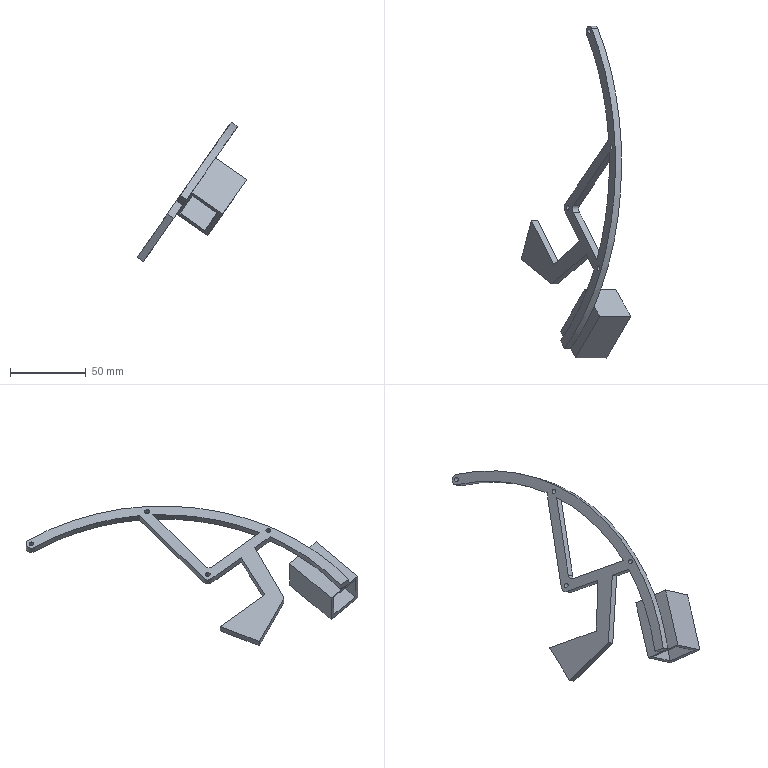Component | NX | LOWER_LEG | 1 solid | 42 faces | volume 29332 mm3 | plane 28 | cylinder 14 | commonest cylinder face diameters 3 x6 300 x3 8.286 x1 7 x1 314 x1 6.571 x1 20 x1